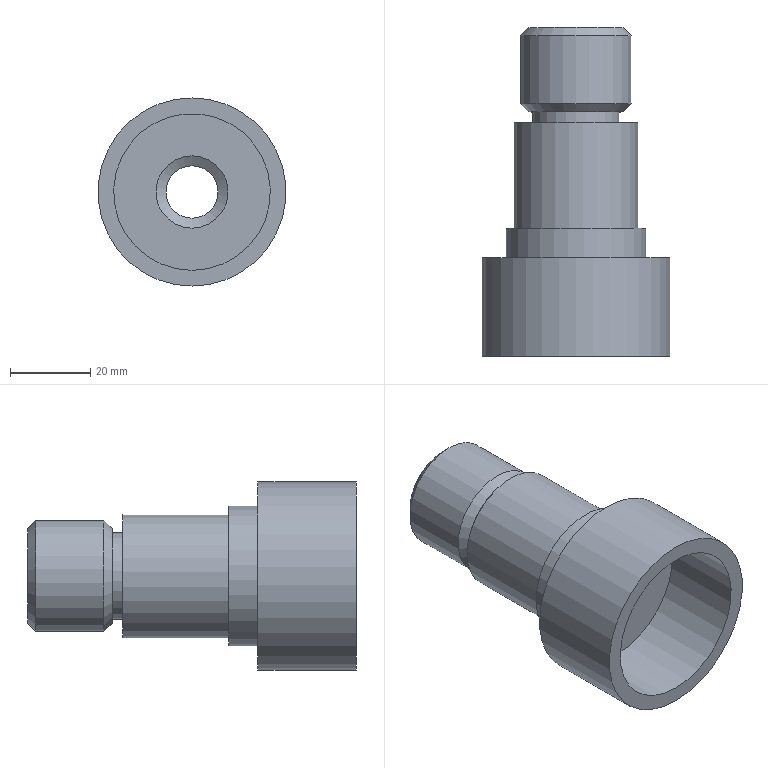Component | NX | VENT_VALVE | 1 solid | 18 faces | box 46.8 x 81.8 x 46.8 mm | volume 45200 mm3 | cylinder 8 | plane 7 | cone 3 | commonest cylinder face diameters 30.8 x1 34.8 x1 46.8 x1 39 x1 13 x1 27.592 x1 21.592 x1 18 x1
STEP:
#1=CARTESIAN_POINT('',(0.,0.,0.));
#2=DIRECTION('',(0.,0.,1.));
#3=DIRECTION('',(1.,0.,0.));
#4=AXIS2_PLACEMENT_3D('',#1,#2,#3);
#5=CARTESIAN_POINT('',(43.195,100.209,-15.4));
#6=VERTEX_POINT('',#5);
#7=CARTESIAN_POINT('',(43.195,100.209,0.));
#8=DIRECTION('',(0.,-1.,0.));
#9=DIRECTION('',(0.,0.,-1.));
#10=AXIS2_PLACEMENT_3D('',#7,#8,#9);
#11=CIRCLE('',#10,15.4);
#12=CARTESIAN_POINT('',(43.195,68.409,0.));
#13=DIRECTION('',(0.,-1.,0.));
#14=DIRECTION('',(0.,0.,-1.));
#15=AXIS2_PLACEMENT_3D('',#12,#13,#14);
#16=CYLINDRICAL_SURFACE('',#15,15.4);
#17=CARTESIAN_POINT('',(0.,-31.8));
#18=DIRECTION('',(1.,0.));
#19=VECTOR('',#18,1.);
#20=LINE('',#17,#19);
#21=(GEOMETRIC_REPRESENTATION_CONTEXT(2)PARAMETRIC_REPRESENTATION_CONTEXT()REPRESENTATION_CONTEXT('',''));
#22=DEFINITIONAL_REPRESENTATION('',(#20),#21);
#23=PCURVE('',#16,#22);
#24=CARTESIAN_POINT('',(27.795,100.209,0.));
#25=DIRECTION('',(0.,-1.,0.));
#26=DIRECTION('',(0.,0.,-1.));
#27=AXIS2_PLACEMENT_3D('',#24,#25,#26);
#28=PLANE('',#27);
#29=CARTESIAN_POINT('',(0.,15.4));
#30=DIRECTION('',(1.,0.));
#31=AXIS2_PLACEMENT_2D('',#29,#30);
#32=CIRCLE('',#31,15.4);
#33=(GEOMETRIC_REPRESENTATION_CONTEXT(2)PARAMETRIC_REPRESENTATION_CONTEXT()REPRESENTATION_CONTEXT('',''));
#34=DEFINITIONAL_REPRESENTATION('',(#32),#33);
#35=PCURVE('',#28,#34);
#36=SURFACE_CURVE('',#11,(#23,#35),.PCURVE_S1.);
#37=EDGE_CURVE('',#6,#6,#36,.T.);
#38=ORIENTED_EDGE('',*,*,#37,.F.);
#39=CARTESIAN_POINT('',(43.195,126.509,-15.4));
#40=VERTEX_POINT('',#39);
#41=CARTESIAN_POINT('',(43.195,126.509,-15.4));
#42=CARTESIAN_POINT('',(43.195,100.209,-15.4));
#43=B_SPLINE_CURVE_WITH_KNOTS('',1,(#41,#42),.UNSPECIFIED.,.F.,.F.,(2,2),(-58.1,-31.8),.PIECEWISE_BEZIER_KNOTS.);
#44=CARTESIAN_POINT('',(0.,0.));
#45=DIRECTION('',(0.,1.));
#46=VECTOR('',#45,1.);
#47=LINE('',#44,#46);
#48=(GEOMETRIC_REPRESENTATION_CONTEXT(2)PARAMETRIC_REPRESENTATION_CONTEXT()REPRESENTATION_CONTEXT('',''));
#49=DEFINITIONAL_REPRESENTATION('',(#47),#48);
#50=PCURVE('',#16,#49);
#51=CARTESIAN_POINT('',(6.283,0.));
#52=DIRECTION('',(0.,1.));
#53=VECTOR('',#52,1.);
#54=LINE('',#51,#53);
#55=(GEOMETRIC_REPRESENTATION_CONTEXT(2)PARAMETRIC_REPRESENTATION_CONTEXT()REPRESENTATION_CONTEXT('',''));
#56=DEFINITIONAL_REPRESENTATION('',(#54),#55);
#57=PCURVE('',#16,#56);
#58=SEAM_CURVE('',#43,(#50,#57),.PCURVE_S1.);
#59=EDGE_CURVE('',#40,#6,#58,.T.);
#60=ORIENTED_EDGE('',*,*,#59,.F.);
#61=CARTESIAN_POINT('',(43.195,126.509,0.));
#62=DIRECTION('',(0.,-1.,0.));
#63=DIRECTION('',(0.,0.,-1.));
#64=AXIS2_PLACEMENT_3D('',#61,#62,#63);
#65=CIRCLE('',#64,15.4);
#66=CARTESIAN_POINT('',(0.,-58.1));
#67=DIRECTION('',(1.,0.));
#68=VECTOR('',#67,1.);
#69=LINE('',#66,#68);
#70=(GEOMETRIC_REPRESENTATION_CONTEXT(2)PARAMETRIC_REPRESENTATION_CONTEXT()REPRESENTATION_CONTEXT('',''));
#71=DEFINITIONAL_REPRESENTATION('',(#69),#70);
#72=PCURVE('',#16,#71);
#73=CARTESIAN_POINT('',(32.399,126.509,0.));
#74=DIRECTION('',(0.,-1.,0.));
#75=DIRECTION('',(0.,0.,-1.));
#76=AXIS2_PLACEMENT_3D('',#73,#74,#75);
#77=PLANE('',#76);
#78=CARTESIAN_POINT('',(0.,10.796));
#79=DIRECTION('',(1.,0.));
#80=AXIS2_PLACEMENT_2D('',#78,#79);
#81=CIRCLE('',#80,15.4);
#82=(GEOMETRIC_REPRESENTATION_CONTEXT(2)PARAMETRIC_REPRESENTATION_CONTEXT()REPRESENTATION_CONTEXT('',''));
#83=DEFINITIONAL_REPRESENTATION('',(#81),#82);
#84=PCURVE('',#77,#83);
#85=SURFACE_CURVE('',#65,(#72,#84),.PCURVE_S1.);
#86=EDGE_CURVE('',#40,#40,#85,.T.);
#87=ORIENTED_EDGE('',*,*,#86,.T.);
#88=ORIENTED_EDGE('',*,*,#59,.T.);
#89=EDGE_LOOP('',(#38,#60,#87,#88));
#90=FACE_BOUND('',#89,.T.);
#91=ADVANCED_FACE('',(#90),#16,.T.);
#92=CARTESIAN_POINT('',(43.195,100.209,-17.4));
#93=VERTEX_POINT('',#92);
#94=CARTESIAN_POINT('',(43.195,100.209,0.));
#95=DIRECTION('',(0.,-1.,0.));
#96=DIRECTION('',(0.,0.,-1.));
#97=AXIS2_PLACEMENT_3D('',#94,#95,#96);
#98=CIRCLE('',#97,17.4);
#99=CARTESIAN_POINT('',(0.,15.4));
#100=DIRECTION('',(1.,0.));
#101=AXIS2_PLACEMENT_2D('',#99,#100);
#102=CIRCLE('',#101,17.4);
#103=(GEOMETRIC_REPRESENTATION_CONTEXT(2)PARAMETRIC_REPRESENTATION_CONTEXT()REPRESENTATION_CONTEXT('',''));
#104=DEFINITIONAL_REPRESENTATION('',(#102),#103);
#105=PCURVE('',#28,#104);
#106=CARTESIAN_POINT('',(43.195,68.409,0.));
#107=DIRECTION('',(0.,-1.,0.));
#108=DIRECTION('',(0.,0.,-1.));
#109=AXIS2_PLACEMENT_3D('',#106,#107,#108);
#110=CYLINDRICAL_SURFACE('',#109,17.4);
#111=CARTESIAN_POINT('',(0.,-31.8));
#112=DIRECTION('',(1.,0.));
#113=VECTOR('',#112,1.);
#114=LINE('',#111,#113);
#115=(GEOMETRIC_REPRESENTATION_CONTEXT(2)PARAMETRIC_REPRESENTATION_CONTEXT()REPRESENTATION_CONTEXT('',''));
#116=DEFINITIONAL_REPRESENTATION('',(#114),#115);
#117=PCURVE('',#110,#116);
#118=SURFACE_CURVE('',#98,(#105,#117),.PCURVE_S1.);
#119=EDGE_CURVE('',#93,#93,#118,.T.);
#120=ORIENTED_EDGE('',*,*,#119,.F.);
#121=EDGE_LOOP('',(#120));
#122=FACE_BOUND('',#121,.T.);
#123=ORIENTED_EDGE('',*,*,#37,.T.);
#124=EDGE_LOOP('',(#123));
#125=FACE_BOUND('',#124,.T.);
#126=ADVANCED_FACE('',(#122,#125),#28,.F.);
#127=CARTESIAN_POINT('',(43.195,92.909,-17.4));
#128=VERTEX_POINT('',#127);
#129=CARTESIAN_POINT('',(43.195,92.909,0.));
#130=DIRECTION('',(0.,-1.,0.));
#131=DIRECTION('',(0.,0.,-1.));
#132=AXIS2_PLACEMENT_3D('',#129,#130,#131);
#133=CIRCLE('',#132,17.4);
#134=CARTESIAN_POINT('',(0.,-24.5));
#135=DIRECTION('',(1.,0.));
#136=VECTOR('',#135,1.);
#137=LINE('',#134,#136);
#138=(GEOMETRIC_REPRESENTATION_CONTEXT(2)PARAMETRIC_REPRESENTATION_CONTEXT()REPRESENTATION_CONTEXT('',''));
#139=DEFINITIONAL_REPRESENTATION('',(#137),#138);
#140=PCURVE('',#110,#139);
#141=CARTESIAN_POINT('',(25.795,92.909,0.));
#142=DIRECTION('',(0.,-1.,0.));
#143=DIRECTION('',(0.,0.,-1.));
#144=AXIS2_PLACEMENT_3D('',#141,#142,#143);
#145=PLANE('',#144);
#146=CARTESIAN_POINT('',(0.,17.4));
#147=DIRECTION('',(1.,0.));
#148=AXIS2_PLACEMENT_2D('',#146,#147);
#149=CIRCLE('',#148,17.4);
#150=(GEOMETRIC_REPRESENTATION_CONTEXT(2)PARAMETRIC_REPRESENTATION_CONTEXT()REPRESENTATION_CONTEXT('',''));
#151=DEFINITIONAL_REPRESENTATION('',(#149),#150);
#152=PCURVE('',#145,#151);
#153=SURFACE_CURVE('',#133,(#140,#152),.PCURVE_S1.);
#154=EDGE_CURVE('',#128,#128,#153,.T.);
#155=ORIENTED_EDGE('',*,*,#154,.F.);
#156=CARTESIAN_POINT('',(43.195,100.209,-17.4));
#157=CARTESIAN_POINT('',(43.195,92.909,-17.4));
#158=B_SPLINE_CURVE_WITH_KNOTS('',1,(#156,#157),.UNSPECIFIED.,.F.,.F.,(2,2),(-31.8,-24.5),.PIECEWISE_BEZIER_KNOTS.);
#159=CARTESIAN_POINT('',(0.,0.));
#160=DIRECTION('',(0.,1.));
#161=VECTOR('',#160,1.);
#162=LINE('',#159,#161);
#163=(GEOMETRIC_REPRESENTATION_CONTEXT(2)PARAMETRIC_REPRESENTATION_CONTEXT()REPRESENTATION_CONTEXT('',''));
#164=DEFINITIONAL_REPRESENTATION('',(#162),#163);
#165=PCURVE('',#110,#164);
#166=CARTESIAN_POINT('',(6.283,0.));
#167=DIRECTION('',(0.,1.));
#168=VECTOR('',#167,1.);
#169=LINE('',#166,#168);
#170=(GEOMETRIC_REPRESENTATION_CONTEXT(2)PARAMETRIC_REPRESENTATION_CONTEXT()REPRESENTATION_CONTEXT('',''));
#171=DEFINITIONAL_REPRESENTATION('',(#169),#170);
#172=PCURVE('',#110,#171);
#173=SEAM_CURVE('',#158,(#165,#172),.PCURVE_S1.);
#174=EDGE_CURVE('',#93,#128,#173,.T.);
#175=ORIENTED_EDGE('',*,*,#174,.F.);
#176=ORIENTED_EDGE('',*,*,#119,.T.);
#177=ORIENTED_EDGE('',*,*,#174,.T.);
#178=EDGE_LOOP('',(#155,#175,#176,#177));
#179=FACE_BOUND('',#178,.T.);
#180=ADVANCED_FACE('',(#179),#110,.T.);
#181=CARTESIAN_POINT('',(43.195,92.909,-23.4));
#182=VERTEX_POINT('',#181);
#183=CARTESIAN_POINT('',(43.195,92.909,0.));
#184=DIRECTION('',(0.,-1.,0.));
#185=DIRECTION('',(0.,0.,-1.));
#186=AXIS2_PLACEMENT_3D('',#183,#184,#185);
#187=CIRCLE('',#186,23.4);
#188=CARTESIAN_POINT('',(0.,17.4));
#189=DIRECTION('',(1.,0.));
#190=AXIS2_PLACEMENT_2D('',#188,#189);
#191=CIRCLE('',#190,23.4);
#192=(GEOMETRIC_REPRESENTATION_CONTEXT(2)PARAMETRIC_REPRESENTATION_CONTEXT()REPRESENTATION_CONTEXT('',''));
#193=DEFINITIONAL_REPRESENTATION('',(#191),#192);
#194=PCURVE('',#145,#193);
#195=CARTESIAN_POINT('',(43.195,68.409,0.));
#196=DIRECTION('',(0.,-1.,0.));
#197=DIRECTION('',(0.,0.,-1.));
#198=AXIS2_PLACEMENT_3D('',#195,#196,#197);
#199=CYLINDRICAL_SURFACE('',#198,23.4);
#200=CARTESIAN_POINT('',(0.,-24.5));
#201=DIRECTION('',(1.,0.));
#202=VECTOR('',#201,1.);
#203=LINE('',#200,#202);
#204=(GEOMETRIC_REPRESENTATION_CONTEXT(2)PARAMETRIC_REPRESENTATION_CONTEXT()REPRESENTATION_CONTEXT('',''));
#205=DEFINITIONAL_REPRESENTATION('',(#203),#204);
#206=PCURVE('',#199,#205);
#207=SURFACE_CURVE('',#187,(#194,#206),.PCURVE_S1.);
#208=EDGE_CURVE('',#182,#182,#207,.T.);
#209=ORIENTED_EDGE('',*,*,#208,.F.);
#210=EDGE_LOOP('',(#209));
#211=FACE_BOUND('',#210,.T.);
#212=ORIENTED_EDGE('',*,*,#154,.T.);
#213=EDGE_LOOP('',(#212));
#214=FACE_BOUND('',#213,.T.);
#215=ADVANCED_FACE('',(#211,#214),#145,.F.);
#216=CARTESIAN_POINT('',(43.195,68.409,-23.4));
#217=VERTEX_POINT('',#216);
#218=CARTESIAN_POINT('',(43.195,68.409,0.));
#219=DIRECTION('',(0.,-1.,0.));
#220=DIRECTION('',(0.,0.,-1.));
#221=AXIS2_PLACEMENT_3D('',#218,#219,#220);
#222=CIRCLE('',#221,23.4);
#223=CARTESIAN_POINT('',(0.,0.));
#224=DIRECTION('',(1.,0.));
#225=VECTOR('',#224,1.);
#226=LINE('',#223,#225);
#227=(GEOMETRIC_REPRESENTATION_CONTEXT(2)PARAMETRIC_REPRESENTATION_CONTEXT()REPRESENTATION_CONTEXT('',''));
#228=DEFINITIONAL_REPRESENTATION('',(#226),#227);
#229=PCURVE('',#199,#228);
#230=CARTESIAN_POINT('',(19.795,68.409,0.));
#231=DIRECTION('',(0.,1.,0.));
#232=DIRECTION('',(0.,0.,1.));
#233=AXIS2_PLACEMENT_3D('',#230,#231,#232);
#234=PLANE('',#233);
#235=CARTESIAN_POINT('',(-23.4,23.4));
#236=CARTESIAN_POINT('',(-23.4,63.93));
#237=CARTESIAN_POINT('',(11.7,43.665));
#238=CARTESIAN_POINT('',(46.8,23.4));
#239=CARTESIAN_POINT('',(11.7,3.135));
#240=CARTESIAN_POINT('',(-23.4,-17.13));
#241=CARTESIAN_POINT('',(-23.4,23.4));
#242=(BOUNDED_CURVE()B_SPLINE_CURVE(2,(#235,#236,#237,#238,#239,#240,#241),.UNSPECIFIED.,.T.,.F.)B_SPLINE_CURVE_WITH_KNOTS((1,2,2,2,2,1),(-2.094,0.,2.094,4.189,6.283,8.378),.UNSPECIFIED.)CURVE()GEOMETRIC_REPRESENTATION_ITEM()RATIONAL_B_SPLINE_CURVE((1.,0.5,1.,0.5,1.,0.5,1.))REPRESENTATION_ITEM(''));
#243=(GEOMETRIC_REPRESENTATION_CONTEXT(2)PARAMETRIC_REPRESENTATION_CONTEXT()REPRESENTATION_CONTEXT('',''));
#244=DEFINITIONAL_REPRESENTATION('',(#242),#243);
#245=PCURVE('',#234,#244);
#246=SURFACE_CURVE('',#222,(#229,#245),.PCURVE_S1.);
#247=EDGE_CURVE('',#217,#217,#246,.T.);
#248=ORIENTED_EDGE('',*,*,#247,.F.);
#249=CARTESIAN_POINT('',(43.195,92.909,-23.4));
#250=CARTESIAN_POINT('',(43.195,68.409,-23.4));
#251=B_SPLINE_CURVE_WITH_KNOTS('',1,(#249,#250),.UNSPECIFIED.,.F.,.F.,(2,2),(-24.5,0.),.PIECEWISE_BEZIER_KNOTS.);
#252=CARTESIAN_POINT('',(0.,0.));
#253=DIRECTION('',(0.,1.));
#254=VECTOR('',#253,1.);
#255=LINE('',#252,#254);
#256=(GEOMETRIC_REPRESENTATION_CONTEXT(2)PARAMETRIC_REPRESENTATION_CONTEXT()REPRESENTATION_CONTEXT('',''));
#257=DEFINITIONAL_REPRESENTATION('',(#255),#256);
#258=PCURVE('',#199,#257);
#259=CARTESIAN_POINT('',(6.283,0.));
#260=DIRECTION('',(0.,1.));
#261=VECTOR('',#260,1.);
#262=LINE('',#259,#261);
#263=(GEOMETRIC_REPRESENTATION_CONTEXT(2)PARAMETRIC_REPRESENTATION_CONTEXT()REPRESENTATION_CONTEXT('',''));
#264=DEFINITIONAL_REPRESENTATION('',(#262),#263);
#265=PCURVE('',#199,#264);
#266=SEAM_CURVE('',#251,(#258,#265),.PCURVE_S1.);
#267=EDGE_CURVE('',#182,#217,#266,.T.);
#268=ORIENTED_EDGE('',*,*,#267,.F.);
#269=ORIENTED_EDGE('',*,*,#208,.T.);
#270=ORIENTED_EDGE('',*,*,#267,.T.);
#271=EDGE_LOOP('',(#248,#268,#269,#270));
#272=FACE_BOUND('',#271,.T.);
#273=ADVANCED_FACE('',(#272),#199,.T.);
#274=CARTESIAN_POINT('',(43.195,68.409,-19.5));
#275=VERTEX_POINT('',#274);
#276=CARTESIAN_POINT('',(43.195,68.409,0.));
#277=DIRECTION('',(0.,-1.,0.));
#278=DIRECTION('',(0.,0.,-1.));
#279=AXIS2_PLACEMENT_3D('',#276,#277,#278);
#280=CIRCLE('',#279,19.5);
#281=CARTESIAN_POINT('',(-19.5,23.4));
#282=CARTESIAN_POINT('',(-19.5,57.175));
#283=CARTESIAN_POINT('',(9.75,40.287));
#284=CARTESIAN_POINT('',(39.,23.4));
#285=CARTESIAN_POINT('',(9.75,6.513));
#286=CARTESIAN_POINT('',(-19.5,-10.375));
#287=CARTESIAN_POINT('',(-19.5,23.4));
#288=(BOUNDED_CURVE()B_SPLINE_CURVE(2,(#281,#282,#283,#284,#285,#286,#287),.UNSPECIFIED.,.T.,.F.)B_SPLINE_CURVE_WITH_KNOTS((1,2,2,2,2,1),(-2.094,0.,2.094,4.189,6.283,8.378),.UNSPECIFIED.)CURVE()GEOMETRIC_REPRESENTATION_ITEM()RATIONAL_B_SPLINE_CURVE((1.,0.5,1.,0.5,1.,0.5,1.))REPRESENTATION_ITEM(''));
#289=(GEOMETRIC_REPRESENTATION_CONTEXT(2)PARAMETRIC_REPRESENTATION_CONTEXT()REPRESENTATION_CONTEXT('',''));
#290=DEFINITIONAL_REPRESENTATION('',(#288),#289);
#291=PCURVE('',#234,#290);
#292=CARTESIAN_POINT('',(43.195,68.409,0.));
#293=DIRECTION('',(0.,-1.,0.));
#294=DIRECTION('',(0.,0.,-1.));
#295=AXIS2_PLACEMENT_3D('',#292,#293,#294);
#296=CYLINDRICAL_SURFACE('',#295,19.5);
#297=CARTESIAN_POINT('',(0.,0.));
#298=DIRECTION('',(1.,0.));
#299=VECTOR('',#298,1.);
#300=LINE('',#297,#299);
#301=(GEOMETRIC_REPRESENTATION_CONTEXT(2)PARAMETRIC_REPRESENTATION_CONTEXT()REPRESENTATION_CONTEXT('',''));
#302=DEFINITIONAL_REPRESENTATION('',(#300),#301);
#303=PCURVE('',#296,#302);
#304=SURFACE_CURVE('',#280,(#291,#303),.PCURVE_S1.);
#305=EDGE_CURVE('',#275,#275,#304,.T.);
#306=ORIENTED_EDGE('',*,*,#305,.F.);
#307=EDGE_LOOP('',(#306));
#308=FACE_BOUND('',#307,.T.);
#309=ORIENTED_EDGE('',*,*,#247,.T.);
#310=EDGE_LOOP('',(#309));
#311=FACE_BOUND('',#310,.T.);
#312=ADVANCED_FACE('',(#308,#311),#234,.F.);
#313=CARTESIAN_POINT('',(43.195,89.109,-19.5));
#314=VERTEX_POINT('',#313);
#315=CARTESIAN_POINT('',(43.195,89.109,0.));
#316=DIRECTION('',(0.,-1.,0.));
#317=DIRECTION('',(0.,0.,-1.));
#318=AXIS2_PLACEMENT_3D('',#315,#316,#317);
#319=CIRCLE('',#318,19.5);
#320=CARTESIAN_POINT('',(0.,-20.7));
#321=DIRECTION('',(1.,0.));
#322=VECTOR('',#321,1.);
#323=LINE('',#320,#322);
#324=(GEOMETRIC_REPRESENTATION_CONTEXT(2)PARAMETRIC_REPRESENTATION_CONTEXT()REPRESENTATION_CONTEXT('',''));
#325=DEFINITIONAL_REPRESENTATION('',(#323),#324);
#326=PCURVE('',#296,#325);
#327=CARTESIAN_POINT('',(23.695,89.109,0.));
#328=DIRECTION('',(0.,1.,0.));
#329=DIRECTION('',(0.,0.,1.));
#330=AXIS2_PLACEMENT_3D('',#327,#328,#329);
#331=PLANE('',#330);
#332=CARTESIAN_POINT('',(-19.5,19.5));
#333=CARTESIAN_POINT('',(-19.5,53.275));
#334=CARTESIAN_POINT('',(9.75,36.387));
#335=CARTESIAN_POINT('',(39.,19.5));
#336=CARTESIAN_POINT('',(9.75,2.613));
#337=CARTESIAN_POINT('',(-19.5,-14.275));
#338=CARTESIAN_POINT('',(-19.5,19.5));
#339=(BOUNDED_CURVE()B_SPLINE_CURVE(2,(#332,#333,#334,#335,#336,#337,#338),.UNSPECIFIED.,.T.,.F.)B_SPLINE_CURVE_WITH_KNOTS((1,2,2,2,2,1),(-2.094,0.,2.094,4.189,6.283,8.378),.UNSPECIFIED.)CURVE()GEOMETRIC_REPRESENTATION_ITEM()RATIONAL_B_SPLINE_CURVE((1.,0.5,1.,0.5,1.,0.5,1.))REPRESENTATION_ITEM(''));
#340=(GEOMETRIC_REPRESENTATION_CONTEXT(2)PARAMETRIC_REPRESENTATION_CONTEXT()REPRESENTATION_CONTEXT('',''));
#341=DEFINITIONAL_REPRESENTATION('',(#339),#340);
#342=PCURVE('',#331,#341);
#343=SURFACE_CURVE('',#319,(#326,#342),.PCURVE_S1.);
#344=EDGE_CURVE('',#314,#314,#343,.T.);
#345=ORIENTED_EDGE('',*,*,#344,.T.);
#346=CARTESIAN_POINT('',(43.195,89.109,-19.5));
#347=CARTESIAN_POINT('',(43.195,68.409,-19.5));
#348=B_SPLINE_CURVE_WITH_KNOTS('',1,(#346,#347),.UNSPECIFIED.,.F.,.F.,(2,2),(-20.7,0.),.PIECEWISE_BEZIER_KNOTS.);
#349=CARTESIAN_POINT('',(6.283,0.));
#350=DIRECTION('',(0.,1.));
#351=VECTOR('',#350,1.);
#352=LINE('',#349,#351);
#353=(GEOMETRIC_REPRESENTATION_CONTEXT(2)PARAMETRIC_REPRESENTATION_CONTEXT()REPRESENTATION_CONTEXT('',''));
#354=DEFINITIONAL_REPRESENTATION('',(#352),#353);
#355=PCURVE('',#296,#354);
#356=CARTESIAN_POINT('',(0.,0.));
#357=DIRECTION('',(0.,1.));
#358=VECTOR('',#357,1.);
#359=LINE('',#356,#358);
#360=(GEOMETRIC_REPRESENTATION_CONTEXT(2)PARAMETRIC_REPRESENTATION_CONTEXT()REPRESENTATION_CONTEXT('',''));
#361=DEFINITIONAL_REPRESENTATION('',(#359),#360);
#362=PCURVE('',#296,#361);
#363=SEAM_CURVE('',#348,(#355,#362),.PCURVE_S1.);
#364=EDGE_CURVE('',#314,#275,#363,.T.);
#365=ORIENTED_EDGE('',*,*,#364,.T.);
#366=ORIENTED_EDGE('',*,*,#305,.F.);
#367=ORIENTED_EDGE('',*,*,#364,.F.);
#368=EDGE_LOOP('',(#345,#365,#366,#367));
#369=FACE_BOUND('',#368,.F.);
#370=ADVANCED_FACE('',(#369),#296,.F.);
#371=CARTESIAN_POINT('',(43.195,89.109,9.));
#372=VERTEX_POINT('',#371);
#373=CARTESIAN_POINT('',(43.195,89.109,0.));
#374=DIRECTION('',(0.,1.,0.));
#375=DIRECTION('',(0.,0.,1.));
#376=AXIS2_PLACEMENT_3D('',#373,#374,#375);
#377=CIRCLE('',#376,9.);
#378=CARTESIAN_POINT('',(0.,19.5));
#379=DIRECTION('',(1.,0.));
#380=AXIS2_PLACEMENT_2D('',#378,#379);
#381=CIRCLE('',#380,9.);
#382=(GEOMETRIC_REPRESENTATION_CONTEXT(2)PARAMETRIC_REPRESENTATION_CONTEXT()REPRESENTATION_CONTEXT('',''));
#383=DEFINITIONAL_REPRESENTATION('',(#381),#382);
#384=PCURVE('',#331,#383);
#385=CARTESIAN_POINT('',(43.195,89.109,0.));
#386=DIRECTION('',(0.,1.,0.));
#387=DIRECTION('',(0.,0.,1.));
#388=AXIS2_PLACEMENT_3D('',#385,#386,#387);
#389=CYLINDRICAL_SURFACE('',#388,9.);
#390=CARTESIAN_POINT('',(0.,0.));
#391=DIRECTION('',(1.,0.));
#392=VECTOR('',#391,1.);
#393=LINE('',#390,#392);
#394=(GEOMETRIC_REPRESENTATION_CONTEXT(2)PARAMETRIC_REPRESENTATION_CONTEXT()REPRESENTATION_CONTEXT('',''));
#395=DEFINITIONAL_REPRESENTATION('',(#393),#394);
#396=PCURVE('',#389,#395);
#397=SURFACE_CURVE('',#377,(#384,#396),.PCURVE_S1.);
#398=EDGE_CURVE('',#372,#372,#397,.T.);
#399=ORIENTED_EDGE('',*,*,#398,.T.);
#400=EDGE_LOOP('',(#399));
#401=FACE_BOUND('',#400,.T.);
#402=ORIENTED_EDGE('',*,*,#344,.T.);
#403=EDGE_LOOP('',(#402));
#404=FACE_BOUND('',#403,.T.);
#405=ADVANCED_FACE('',(#401,#404),#331,.F.);
#406=CARTESIAN_POINT('',(43.195,121.612,-6.5));
#407=VERTEX_POINT('',#406);
#408=CARTESIAN_POINT('',(43.195,121.612,0.));
#409=DIRECTION('',(0.,-1.,0.));
#410=DIRECTION('',(0.,0.,-1.));
#411=AXIS2_PLACEMENT_3D('',#408,#409,#410);
#412=CIRCLE('',#411,6.5);
#413=CARTESIAN_POINT('',(43.195,68.409,0.));
#414=DIRECTION('',(0.,-1.,0.));
#415=DIRECTION('',(0.,0.,-1.));
#416=AXIS2_PLACEMENT_3D('',#413,#414,#415);
#417=CYLINDRICAL_SURFACE('',#416,6.5);
#418=CARTESIAN_POINT('',(0.,-53.202));
#419=DIRECTION('',(1.,0.));
#420=VECTOR('',#419,1.);
#421=LINE('',#418,#420);
#422=(GEOMETRIC_REPRESENTATION_CONTEXT(2)PARAMETRIC_REPRESENTATION_CONTEXT()REPRESENTATION_CONTEXT('',''));
#423=DEFINITIONAL_REPRESENTATION('',(#421),#422);
#424=PCURVE('',#417,#423);
#425=CARTESIAN_POINT('',(43.195,120.109,0.));
#426=DIRECTION('',(0.,-1.,0.));
#427=DIRECTION('',(0.,0.,-1.));
#428=AXIS2_PLACEMENT_3D('',#425,#426,#427);
#429=CONICAL_SURFACE('',#428,9.,1.03);
#430=CARTESIAN_POINT('',(0.,-1.502));
#431=DIRECTION('',(1.,0.));
#432=VECTOR('',#431,1.);
#433=LINE('',#430,#432);
#434=(GEOMETRIC_REPRESENTATION_CONTEXT(2)PARAMETRIC_REPRESENTATION_CONTEXT()REPRESENTATION_CONTEXT('',''));
#435=DEFINITIONAL_REPRESENTATION('',(#433),#434);
#436=PCURVE('',#429,#435);
#437=SURFACE_CURVE('',#412,(#424,#436),.PCURVE_S1.);
#438=EDGE_CURVE('',#407,#407,#437,.T.);
#439=ORIENTED_EDGE('',*,*,#438,.F.);
#440=CARTESIAN_POINT('',(43.195,150.209,-6.5));
#441=VERTEX_POINT('',#440);
#442=CARTESIAN_POINT('',(43.195,150.209,-6.5));
#443=CARTESIAN_POINT('',(43.195,121.612,-6.5));
#444=B_SPLINE_CURVE_WITH_KNOTS('',1,(#442,#443),.UNSPECIFIED.,.F.,.F.,(2,2),(-81.8,-53.202),.PIECEWISE_BEZIER_KNOTS.);
#445=CARTESIAN_POINT('',(0.,0.));
#446=DIRECTION('',(0.,1.));
#447=VECTOR('',#446,1.);
#448=LINE('',#445,#447);
#449=(GEOMETRIC_REPRESENTATION_CONTEXT(2)PARAMETRIC_REPRESENTATION_CONTEXT()REPRESENTATION_CONTEXT('',''));
#450=DEFINITIONAL_REPRESENTATION('',(#448),#449);
#451=PCURVE('',#417,#450);
#452=CARTESIAN_POINT('',(6.283,0.));
#453=DIRECTION('',(0.,1.));
#454=VECTOR('',#453,1.);
#455=LINE('',#452,#454);
#456=(GEOMETRIC_REPRESENTATION_CONTEXT(2)PARAMETRIC_REPRESENTATION_CONTEXT()REPRESENTATION_CONTEXT('',''));
#457=DEFINITIONAL_REPRESENTATION('',(#455),#456);
#458=PCURVE('',#417,#457);
#459=SEAM_CURVE('',#444,(#451,#458),.PCURVE_S1.);
#460=EDGE_CURVE('',#441,#407,#459,.T.);
#461=ORIENTED_EDGE('',*,*,#460,.F.);
#462=CARTESIAN_POINT('',(43.195,150.209,0.));
#463=DIRECTION('',(0.,-1.,0.));
#464=DIRECTION('',(0.,0.,-1.));
#465=AXIS2_PLACEMENT_3D('',#462,#463,#464);
#466=CIRCLE('',#465,6.5);
#467=CARTESIAN_POINT('',(0.,-81.8));
#468=DIRECTION('',(1.,0.));
#469=VECTOR('',#468,1.);
#470=LINE('',#467,#469);
#471=(GEOMETRIC_REPRESENTATION_CONTEXT(2)PARAMETRIC_REPRESENTATION_CONTEXT()REPRESENTATION_CONTEXT('',''));
#472=DEFINITIONAL_REPRESENTATION('',(#470),#471);
#473=PCURVE('',#417,#472);
#474=CARTESIAN_POINT('',(36.695,150.209,0.));
#475=DIRECTION('',(0.,-1.,0.));
#476=DIRECTION('',(0.,0.,-1.));
#477=AXIS2_PLACEMENT_3D('',#474,#475,#476);
#478=PLANE('',#477);
#479=CARTESIAN_POINT('',(0.,6.5));
#480=DIRECTION('',(1.,0.));
#481=AXIS2_PLACEMENT_2D('',#479,#480);
#482=CIRCLE('',#481,6.5);
#483=(GEOMETRIC_REPRESENTATION_CONTEXT(2)PARAMETRIC_REPRESENTATION_CONTEXT()REPRESENTATION_CONTEXT('',''));
#484=DEFINITIONAL_REPRESENTATION('',(#482),#483);
#485=PCURVE('',#478,#484);
#486=SURFACE_CURVE('',#466,(#473,#485),.PCURVE_S1.);
#487=EDGE_CURVE('',#441,#441,#486,.T.);
#488=ORIENTED_EDGE('',*,*,#487,.T.);
#489=ORIENTED_EDGE('',*,*,#460,.T.);
#490=EDGE_LOOP('',(#439,#461,#488,#489));
#491=FACE_BOUND('',#490,.F.);
#492=ADVANCED_FACE('',(#491),#417,.F.);
#493=CARTESIAN_POINT('',(43.195,150.209,-11.796));
#494=VERTEX_POINT('',#493);
#495=CARTESIAN_POINT('',(43.195,150.209,0.));
#496=DIRECTION('',(0.,1.,0.));
#497=DIRECTION('',(0.,0.,-1.));
#498=AXIS2_PLACEMENT_3D('',#495,#496,#497);
#499=CIRCLE('',#498,11.796);
#500=CARTESIAN_POINT('',(11.796,6.5));
#501=CARTESIAN_POINT('',(11.796,-13.931));
#502=CARTESIAN_POINT('',(-5.898,-3.716));
#503=CARTESIAN_POINT('',(-23.592,6.5));
#504=CARTESIAN_POINT('',(-5.898,16.716));
#505=CARTESIAN_POINT('',(11.796,26.931));
#506=CARTESIAN_POINT('',(11.796,6.5));
#507=(BOUNDED_CURVE()B_SPLINE_CURVE(2,(#500,#501,#502,#503,#504,#505,#506),.UNSPECIFIED.,.T.,.F.)B_SPLINE_CURVE_WITH_KNOTS((1,2,2,2,2,1),(-2.094,0.,2.094,4.189,6.283,8.378),.UNSPECIFIED.)CURVE()GEOMETRIC_REPRESENTATION_ITEM()RATIONAL_B_SPLINE_CURVE((1.,0.5,1.,0.5,1.,0.5,1.))REPRESENTATION_ITEM(''));
#508=(GEOMETRIC_REPRESENTATION_CONTEXT(2)PARAMETRIC_REPRESENTATION_CONTEXT()REPRESENTATION_CONTEXT('',''));
#509=DEFINITIONAL_REPRESENTATION('',(#507),#508);
#510=PCURVE('',#478,#509);
#511=CARTESIAN_POINT('',(43.195,148.209,0.));
#512=DIRECTION('',(0.,-1.,0.));
#513=DIRECTION('',(0.,0.,-1.));
#514=AXIS2_PLACEMENT_3D('',#511,#512,#513);
#515=CONICAL_SURFACE('',#514,13.796,0.7854);
#516=CARTESIAN_POINT('',(6.283,-2.));
#517=DIRECTION('',(-1.,0.));
#518=VECTOR('',#517,1.);
#519=LINE('',#516,#518);
#520=(GEOMETRIC_REPRESENTATION_CONTEXT(2)PARAMETRIC_REPRESENTATION_CONTEXT()REPRESENTATION_CONTEXT('',''));
#521=DEFINITIONAL_REPRESENTATION('',(#519),#520);
#522=PCURVE('',#515,#521);
#523=SURFACE_CURVE('',#499,(#510,#522),.PCURVE_S1.);
#524=EDGE_CURVE('',#494,#494,#523,.T.);
#525=ORIENTED_EDGE('',*,*,#524,.T.);
#526=EDGE_LOOP('',(#525));
#527=FACE_BOUND('',#526,.T.);
#528=ORIENTED_EDGE('',*,*,#487,.T.);
#529=EDGE_LOOP('',(#528));
#530=FACE_BOUND('',#529,.T.);
#531=ADVANCED_FACE('',(#527,#530),#478,.F.);
#532=CARTESIAN_POINT('',(43.195,131.209,13.796));
#533=VERTEX_POINT('',#532);
#534=CARTESIAN_POINT('',(43.195,131.209,-13.796));
#535=VERTEX_POINT('',#534);
#536=CARTESIAN_POINT('',(43.195,131.209,0.));
#537=DIRECTION('',(0.,1.,0.));
#538=DIRECTION('',(0.,0.,1.));
#539=AXIS2_PLACEMENT_3D('',#536,#537,#538);
#540=CIRCLE('',#539,13.796);
#541=CARTESIAN_POINT('',(43.195,68.409,0.));
#542=DIRECTION('',(0.,-1.,0.));
#543=DIRECTION('',(0.,0.,-1.));
#544=AXIS2_PLACEMENT_3D('',#541,#542,#543);
#545=CYLINDRICAL_SURFACE('',#544,13.796);
#546=CARTESIAN_POINT('',(3.142,-62.8));
#547=DIRECTION('',(-1.,0.));
#548=VECTOR('',#547,1.);
#549=LINE('',#546,#548);
#550=(GEOMETRIC_REPRESENTATION_CONTEXT(2)PARAMETRIC_REPRESENTATION_CONTEXT()REPRESENTATION_CONTEXT('',''));
#551=DEFINITIONAL_REPRESENTATION('',(#549),#550);
#552=PCURVE('',#545,#551);
#553=CARTESIAN_POINT('',(43.195,129.209,0.));
#554=DIRECTION('',(0.,1.,0.));
#555=DIRECTION('',(0.,0.,1.));
#556=AXIS2_PLACEMENT_3D('',#553,#554,#555);
#557=CONICAL_SURFACE('',#556,11.796,0.7854);
#558=CARTESIAN_POINT('',(0.,2.));
#559=DIRECTION('',(1.,0.));
#560=VECTOR('',#559,1.);
#561=LINE('',#558,#560);
#562=(GEOMETRIC_REPRESENTATION_CONTEXT(2)PARAMETRIC_REPRESENTATION_CONTEXT()REPRESENTATION_CONTEXT('',''));
#563=DEFINITIONAL_REPRESENTATION('',(#561),#562);
#564=PCURVE('',#557,#563);
#565=SURFACE_CURVE('',#540,(#552,#564),.PCURVE_S1.);
#566=EDGE_CURVE('',#533,#535,#565,.T.);
#567=ORIENTED_EDGE('',*,*,#566,.T.);
#568=CARTESIAN_POINT('',(43.195,148.209,-13.796));
#569=VERTEX_POINT('',#568);
#570=CARTESIAN_POINT('',(43.195,148.209,-13.796));
#571=CARTESIAN_POINT('',(43.195,131.209,-13.796));
#572=B_SPLINE_CURVE_WITH_KNOTS('',1,(#570,#571),.UNSPECIFIED.,.F.,.F.,(2,2),(-79.8,-62.8),.PIECEWISE_BEZIER_KNOTS.);
#573=CARTESIAN_POINT('',(0.,0.));
#574=DIRECTION('',(0.,1.));
#575=VECTOR('',#574,1.);
#576=LINE('',#573,#575);
#577=(GEOMETRIC_REPRESENTATION_CONTEXT(2)PARAMETRIC_REPRESENTATION_CONTEXT()REPRESENTATION_CONTEXT('',''));
#578=DEFINITIONAL_REPRESENTATION('',(#576),#577);
#579=PCURVE('',#545,#578);
#580=CARTESIAN_POINT('',(6.283,0.));
#581=DIRECTION('',(0.,1.));
#582=VECTOR('',#581,1.);
#583=LINE('',#580,#582);
#584=(GEOMETRIC_REPRESENTATION_CONTEXT(2)PARAMETRIC_REPRESENTATION_CONTEXT()REPRESENTATION_CONTEXT('',''));
#585=DEFINITIONAL_REPRESENTATION('',(#583),#584);
#586=PCURVE('',#545,#585);
#587=SEAM_CURVE('',#572,(#579,#586),.PCURVE_S1.);
#588=EDGE_CURVE('',#569,#535,#587,.T.);
#589=ORIENTED_EDGE('',*,*,#588,.F.);
#590=CARTESIAN_POINT('',(43.195,148.209,0.));
#591=DIRECTION('',(0.,-1.,0.));
#592=DIRECTION('',(0.,0.,-1.));
#593=AXIS2_PLACEMENT_3D('',#590,#591,#592);
#594=CIRCLE('',#593,13.796);
#595=CARTESIAN_POINT('',(0.,-79.8));
#596=DIRECTION('',(1.,0.));
#597=VECTOR('',#596,1.);
#598=LINE('',#595,#597);
#599=(GEOMETRIC_REPRESENTATION_CONTEXT(2)PARAMETRIC_REPRESENTATION_CONTEXT()REPRESENTATION_CONTEXT('',''));
#600=DEFINITIONAL_REPRESENTATION('',(#598),#599);
#601=PCURVE('',#545,#600);
#602=CARTESIAN_POINT('',(0.,0.));
#603=DIRECTION('',(1.,0.));
#604=VECTOR('',#603,1.);
#605=LINE('',#602,#604);
#606=(GEOMETRIC_REPRESENTATION_CONTEXT(2)PARAMETRIC_REPRESENTATION_CONTEXT()REPRESENTATION_CONTEXT('',''));
#607=DEFINITIONAL_REPRESENTATION('',(#605),#606);
#608=PCURVE('',#515,#607);
#609=SURFACE_CURVE('',#594,(#601,#608),.PCURVE_S1.);
#610=EDGE_CURVE('',#569,#569,#609,.T.);
#611=ORIENTED_EDGE('',*,*,#610,.T.);
#612=ORIENTED_EDGE('',*,*,#588,.T.);
#613=CARTESIAN_POINT('',(43.195,131.209,0.));
#614=DIRECTION('',(0.,1.,0.));
#615=DIRECTION('',(0.,0.,1.));
#616=AXIS2_PLACEMENT_3D('',#613,#614,#615);
#617=CIRCLE('',#616,13.796);
#618=CARTESIAN_POINT('',(9.425,-62.8));
#619=DIRECTION('',(-1.,0.));
#620=VECTOR('',#619,1.);
#621=LINE('',#618,#620);
#622=(GEOMETRIC_REPRESENTATION_CONTEXT(2)PARAMETRIC_REPRESENTATION_CONTEXT()REPRESENTATION_CONTEXT('',''));
#623=DEFINITIONAL_REPRESENTATION('',(#621),#622);
#624=PCURVE('',#545,#623);
#625=CARTESIAN_POINT('',(0.,2.));
#626=DIRECTION('',(1.,0.));
#627=VECTOR('',#626,1.);
#628=LINE('',#625,#627);
#629=(GEOMETRIC_REPRESENTATION_CONTEXT(2)PARAMETRIC_REPRESENTATION_CONTEXT()REPRESENTATION_CONTEXT('',''));
#630=DEFINITIONAL_REPRESENTATION('',(#628),#629);
#631=PCURVE('',#557,#630);
#632=SURFACE_CURVE('',#617,(#624,#631),.PCURVE_S1.);
#633=EDGE_CURVE('',#535,#533,#632,.T.);
#634=ORIENTED_EDGE('',*,*,#633,.T.);
#635=EDGE_LOOP('',(#567,#589,#611,#612,#634));
#636=FACE_BOUND('',#635,.T.);
#637=ADVANCED_FACE('',(#636),#545,.T.);
#638=CARTESIAN_POINT('',(43.195,129.209,11.796));
#639=VERTEX_POINT('',#638);
#640=CARTESIAN_POINT('',(43.195,129.209,0.));
#641=DIRECTION('',(0.,-1.,0.));
#642=DIRECTION('',(0.,0.,1.));
#643=AXIS2_PLACEMENT_3D('',#640,#641,#642);
#644=CIRCLE('',#643,11.796);
#645=CARTESIAN_POINT('',(29.399,129.209,0.));
#646=DIRECTION('',(0.,1.,0.));
#647=DIRECTION('',(0.,0.,1.));
#648=AXIS2_PLACEMENT_3D('',#645,#646,#647);
#649=PLANE('',#648);
#650=CARTESIAN_POINT('',(11.796,13.796));
#651=CARTESIAN_POINT('',(11.796,-6.635));
#652=CARTESIAN_POINT('',(-5.898,3.58));
#653=CARTESIAN_POINT('',(-23.592,13.796));
#654=CARTESIAN_POINT('',(-5.898,24.011));
#655=CARTESIAN_POINT('',(11.796,34.227));
#656=CARTESIAN_POINT('',(11.796,13.796));
#657=(BOUNDED_CURVE()B_SPLINE_CURVE(2,(#650,#651,#652,#653,#654,#655,#656),.UNSPECIFIED.,.T.,.F.)B_SPLINE_CURVE_WITH_KNOTS((1,2,2,2,2,1),(-2.094,0.,2.094,4.189,6.283,8.378),.UNSPECIFIED.)CURVE()GEOMETRIC_REPRESENTATION_ITEM()RATIONAL_B_SPLINE_CURVE((1.,0.5,1.,0.5,1.,0.5,1.))REPRESENTATION_ITEM(''));
#658=(GEOMETRIC_REPRESENTATION_CONTEXT(2)PARAMETRIC_REPRESENTATION_CONTEXT()REPRESENTATION_CONTEXT('',''));
#659=DEFINITIONAL_REPRESENTATION('',(#657),#658);
#660=PCURVE('',#649,#659);
#661=CARTESIAN_POINT('',(6.283,0.));
#662=DIRECTION('',(-1.,0.));
#663=VECTOR('',#662,1.);
#664=LINE('',#661,#663);
#665=(GEOMETRIC_REPRESENTATION_CONTEXT(2)PARAMETRIC_REPRESENTATION_CONTEXT()REPRESENTATION_CONTEXT('',''));
#666=DEFINITIONAL_REPRESENTATION('',(#664),#665);
#667=PCURVE('',#557,#666);
#668=SURFACE_CURVE('',#644,(#660,#667),.PCURVE_S1.);
#669=EDGE_CURVE('',#639,#639,#668,.T.);
#670=ORIENTED_EDGE('',*,*,#669,.T.);
#671=EDGE_LOOP('',(#670));
#672=FACE_BOUND('',#671,.T.);
#673=CARTESIAN_POINT('',(43.195,129.209,-10.796));
#674=VERTEX_POINT('',#673);
#675=CARTESIAN_POINT('',(43.195,129.209,0.));
#676=DIRECTION('',(0.,-1.,0.));
#677=DIRECTION('',(0.,0.,-1.));
#678=AXIS2_PLACEMENT_3D('',#675,#676,#677);
#679=CIRCLE('',#678,10.796);
#680=CARTESIAN_POINT('',(-10.796,13.796));
#681=CARTESIAN_POINT('',(-10.796,32.495));
#682=CARTESIAN_POINT('',(5.398,23.145));
#683=CARTESIAN_POINT('',(21.592,13.796));
#684=CARTESIAN_POINT('',(5.398,4.446));
#685=CARTESIAN_POINT('',(-10.796,-4.903));
#686=CARTESIAN_POINT('',(-10.796,13.796));
#687=(BOUNDED_CURVE()B_SPLINE_CURVE(2,(#680,#681,#682,#683,#684,#685,#686),.UNSPECIFIED.,.T.,.F.)B_SPLINE_CURVE_WITH_KNOTS((1,2,2,2,2,1),(-2.094,0.,2.094,4.189,6.283,8.378),.UNSPECIFIED.)CURVE()GEOMETRIC_REPRESENTATION_ITEM()RATIONAL_B_SPLINE_CURVE((1.,0.5,1.,0.5,1.,0.5,1.))REPRESENTATION_ITEM(''));
#688=(GEOMETRIC_REPRESENTATION_CONTEXT(2)PARAMETRIC_REPRESENTATION_CONTEXT()REPRESENTATION_CONTEXT('',''));
#689=DEFINITIONAL_REPRESENTATION('',(#687),#688);
#690=PCURVE('',#649,#689);
#691=CARTESIAN_POINT('',(43.195,68.409,0.));
#692=DIRECTION('',(0.,-1.,0.));
#693=DIRECTION('',(0.,0.,-1.));
#694=AXIS2_PLACEMENT_3D('',#691,#692,#693);
#695=CYLINDRICAL_SURFACE('',#694,10.796);
#696=CARTESIAN_POINT('',(0.,-60.8));
#697=DIRECTION('',(1.,0.));
#698=VECTOR('',#697,1.);
#699=LINE('',#696,#698);
#700=(GEOMETRIC_REPRESENTATION_CONTEXT(2)PARAMETRIC_REPRESENTATION_CONTEXT()REPRESENTATION_CONTEXT('',''));
#701=DEFINITIONAL_REPRESENTATION('',(#699),#700);
#702=PCURVE('',#695,#701);
#703=SURFACE_CURVE('',#679,(#690,#702),.PCURVE_S1.);
#704=EDGE_CURVE('',#674,#674,#703,.T.);
#705=ORIENTED_EDGE('',*,*,#704,.F.);
#706=EDGE_LOOP('',(#705));
#707=FACE_BOUND('',#706,.T.);
#708=ADVANCED_FACE('',(#672,#707),#649,.F.);
#709=CARTESIAN_POINT('',(43.195,126.509,-10.796));
#710=VERTEX_POINT('',#709);
#711=CARTESIAN_POINT('',(43.195,126.509,0.));
#712=DIRECTION('',(0.,-1.,0.));
#713=DIRECTION('',(0.,0.,-1.));
#714=AXIS2_PLACEMENT_3D('',#711,#712,#713);
#715=CIRCLE('',#714,10.796);
#716=CARTESIAN_POINT('',(0.,-58.1));
#717=DIRECTION('',(1.,0.));
#718=VECTOR('',#717,1.);
#719=LINE('',#716,#718);
#720=(GEOMETRIC_REPRESENTATION_CONTEXT(2)PARAMETRIC_REPRESENTATION_CONTEXT()REPRESENTATION_CONTEXT('',''));
#721=DEFINITIONAL_REPRESENTATION('',(#719),#720);
#722=PCURVE('',#695,#721);
#723=CARTESIAN_POINT('',(0.,10.796));
#724=DIRECTION('',(1.,0.));
#725=AXIS2_PLACEMENT_2D('',#723,#724);
#726=CIRCLE('',#725,10.796);
#727=(GEOMETRIC_REPRESENTATION_CONTEXT(2)PARAMETRIC_REPRESENTATION_CONTEXT()REPRESENTATION_CONTEXT('',''));
#728=DEFINITIONAL_REPRESENTATION('',(#726),#727);
#729=PCURVE('',#77,#728);
#730=SURFACE_CURVE('',#715,(#722,#729),.PCURVE_S1.);
#731=EDGE_CURVE('',#710,#710,#730,.T.);
#732=ORIENTED_EDGE('',*,*,#731,.F.);
#733=CARTESIAN_POINT('',(43.195,129.209,-10.796));
#734=CARTESIAN_POINT('',(43.195,126.509,-10.796));
#735=B_SPLINE_CURVE_WITH_KNOTS('',1,(#733,#734),.UNSPECIFIED.,.F.,.F.,(2,2),(-60.8,-58.1),.PIECEWISE_BEZIER_KNOTS.);
#736=CARTESIAN_POINT('',(0.,0.));
#737=DIRECTION('',(0.,1.));
#738=VECTOR('',#737,1.);
#739=LINE('',#736,#738);
#740=(GEOMETRIC_REPRESENTATION_CONTEXT(2)PARAMETRIC_REPRESENTATION_CONTEXT()REPRESENTATION_CONTEXT('',''));
#741=DEFINITIONAL_REPRESENTATION('',(#739),#740);
#742=PCURVE('',#695,#741);
#743=CARTESIAN_POINT('',(6.283,0.));
#744=DIRECTION('',(0.,1.));
#745=VECTOR('',#744,1.);
#746=LINE('',#743,#745);
#747=(GEOMETRIC_REPRESENTATION_CONTEXT(2)PARAMETRIC_REPRESENTATION_CONTEXT()REPRESENTATION_CONTEXT('',''));
#748=DEFINITIONAL_REPRESENTATION('',(#746),#747);
#749=PCURVE('',#695,#748);
#750=SEAM_CURVE('',#735,(#742,#749),.PCURVE_S1.);
#751=EDGE_CURVE('',#674,#710,#750,.T.);
#752=ORIENTED_EDGE('',*,*,#751,.F.);
#753=ORIENTED_EDGE('',*,*,#704,.T.);
#754=ORIENTED_EDGE('',*,*,#751,.T.);
#755=EDGE_LOOP('',(#732,#752,#753,#754));
#756=FACE_BOUND('',#755,.T.);
#757=ADVANCED_FACE('',(#756),#695,.T.);
#758=ORIENTED_EDGE('',*,*,#86,.F.);
#759=EDGE_LOOP('',(#758));
#760=FACE_BOUND('',#759,.T.);
#761=ORIENTED_EDGE('',*,*,#731,.T.);
#762=EDGE_LOOP('',(#761));
#763=FACE_BOUND('',#762,.T.);
#764=ADVANCED_FACE('',(#760,#763),#77,.F.);
#765=CARTESIAN_POINT('',(43.195,120.109,-9.));
#766=VERTEX_POINT('',#765);
#767=CARTESIAN_POINT('',(43.195,120.109,9.));
#768=VERTEX_POINT('',#767);
#769=CARTESIAN_POINT('',(43.195,120.109,0.));
#770=DIRECTION('',(0.,-1.,0.));
#771=DIRECTION('',(0.,0.,1.));
#772=AXIS2_PLACEMENT_3D('',#769,#770,#771);
#773=CIRCLE('',#772,9.);
#774=CARTESIAN_POINT('',(-3.142,0.));
#775=DIRECTION('',(1.,0.));
#776=VECTOR('',#775,1.);
#777=LINE('',#774,#776);
#778=(GEOMETRIC_REPRESENTATION_CONTEXT(2)PARAMETRIC_REPRESENTATION_CONTEXT()REPRESENTATION_CONTEXT('',''));
#779=DEFINITIONAL_REPRESENTATION('',(#777),#778);
#780=PCURVE('',#429,#779);
#781=CARTESIAN_POINT('',(6.283,31.));
#782=DIRECTION('',(-1.,0.));
#783=VECTOR('',#782,1.);
#784=LINE('',#781,#783);
#785=(GEOMETRIC_REPRESENTATION_CONTEXT(2)PARAMETRIC_REPRESENTATION_CONTEXT()REPRESENTATION_CONTEXT('',''));
#786=DEFINITIONAL_REPRESENTATION('',(#784),#785);
#787=PCURVE('',#389,#786);
#788=SURFACE_CURVE('',#773,(#780,#787),.PCURVE_S1.);
#789=EDGE_CURVE('',#766,#768,#788,.T.);
#790=ORIENTED_EDGE('',*,*,#789,.F.);
#791=CARTESIAN_POINT('',(43.195,121.612,-6.5));
#792=CARTESIAN_POINT('',(43.195,120.109,-9.));
#793=B_SPLINE_CURVE_WITH_KNOTS('',1,(#791,#792),.UNSPECIFIED.,.F.,.F.,(2,2),(-2.917,0.),.PIECEWISE_BEZIER_KNOTS.);
#794=CARTESIAN_POINT('',(0.,0.));
#795=DIRECTION('',(0.,1.));
#796=VECTOR('',#795,1.);
#797=LINE('',#794,#796);
#798=(GEOMETRIC_REPRESENTATION_CONTEXT(2)PARAMETRIC_REPRESENTATION_CONTEXT()REPRESENTATION_CONTEXT('',''));
#799=DEFINITIONAL_REPRESENTATION('',(#797),#798);
#800=PCURVE('',#429,#799);
#801=CARTESIAN_POINT('',(6.283,0.));
#802=DIRECTION('',(0.,1.));
#803=VECTOR('',#802,1.);
#804=LINE('',#801,#803);
#805=(GEOMETRIC_REPRESENTATION_CONTEXT(2)PARAMETRIC_REPRESENTATION_CONTEXT()REPRESENTATION_CONTEXT('',''));
#806=DEFINITIONAL_REPRESENTATION('',(#804),#805);
#807=PCURVE('',#429,#806);
#808=SEAM_CURVE('',#793,(#800,#807),.PCURVE_S1.);
#809=EDGE_CURVE('',#407,#766,#808,.T.);
#810=ORIENTED_EDGE('',*,*,#809,.F.);
#811=ORIENTED_EDGE('',*,*,#438,.T.);
#812=ORIENTED_EDGE('',*,*,#809,.T.);
#813=CARTESIAN_POINT('',(43.195,120.109,0.));
#814=DIRECTION('',(0.,-1.,0.));
#815=DIRECTION('',(0.,0.,1.));
#816=AXIS2_PLACEMENT_3D('',#813,#814,#815);
#817=CIRCLE('',#816,9.);
#818=CARTESIAN_POINT('',(3.142,0.));
#819=DIRECTION('',(1.,0.));
#820=VECTOR('',#819,1.);
#821=LINE('',#818,#820);
#822=(GEOMETRIC_REPRESENTATION_CONTEXT(2)PARAMETRIC_REPRESENTATION_CONTEXT()REPRESENTATION_CONTEXT('',''));
#823=DEFINITIONAL_REPRESENTATION('',(#821),#822);
#824=PCURVE('',#429,#823);
#825=CARTESIAN_POINT('',(6.283,31.));
#826=DIRECTION('',(-1.,0.));
#827=VECTOR('',#826,1.);
#828=LINE('',#825,#827);
#829=(GEOMETRIC_REPRESENTATION_CONTEXT(2)PARAMETRIC_REPRESENTATION_CONTEXT()REPRESENTATION_CONTEXT('',''));
#830=DEFINITIONAL_REPRESENTATION('',(#828),#829);
#831=PCURVE('',#389,#830);
#832=SURFACE_CURVE('',#817,(#824,#831),.PCURVE_S1.);
#833=EDGE_CURVE('',#768,#766,#832,.T.);
#834=ORIENTED_EDGE('',*,*,#833,.F.);
#835=EDGE_LOOP('',(#790,#810,#811,#812,#834));
#836=FACE_BOUND('',#835,.F.);
#837=ADVANCED_FACE('',(#836),#429,.F.);
#838=ORIENTED_EDGE('',*,*,#789,.T.);
#839=CARTESIAN_POINT('',(43.195,89.109,9.));
#840=CARTESIAN_POINT('',(43.195,120.109,9.));
#841=B_SPLINE_CURVE_WITH_KNOTS('',1,(#839,#840),.UNSPECIFIED.,.F.,.F.,(2,2),(0.,31.),.PIECEWISE_BEZIER_KNOTS.);
#842=CARTESIAN_POINT('',(0.,0.));
#843=DIRECTION('',(0.,1.));
#844=VECTOR('',#843,1.);
#845=LINE('',#842,#844);
#846=(GEOMETRIC_REPRESENTATION_CONTEXT(2)PARAMETRIC_REPRESENTATION_CONTEXT()REPRESENTATION_CONTEXT('',''));
#847=DEFINITIONAL_REPRESENTATION('',(#845),#846);
#848=PCURVE('',#389,#847);
#849=CARTESIAN_POINT('',(6.283,0.));
#850=DIRECTION('',(0.,1.));
#851=VECTOR('',#850,1.);
#852=LINE('',#849,#851);
#853=(GEOMETRIC_REPRESENTATION_CONTEXT(2)PARAMETRIC_REPRESENTATION_CONTEXT()REPRESENTATION_CONTEXT('',''));
#854=DEFINITIONAL_REPRESENTATION('',(#852),#853);
#855=PCURVE('',#389,#854);
#856=SEAM_CURVE('',#841,(#848,#855),.PCURVE_S1.);
#857=EDGE_CURVE('',#372,#768,#856,.T.);
#858=ORIENTED_EDGE('',*,*,#857,.F.);
#859=ORIENTED_EDGE('',*,*,#398,.T.);
#860=ORIENTED_EDGE('',*,*,#857,.T.);
#861=ORIENTED_EDGE('',*,*,#833,.T.);
#862=EDGE_LOOP('',(#838,#858,#859,#860,#861));
#863=FACE_BOUND('',#862,.F.);
#864=ADVANCED_FACE('',(#863),#389,.F.);
#865=ORIENTED_EDGE('',*,*,#566,.F.);
#866=CARTESIAN_POINT('',(43.195,129.209,11.796));
#867=CARTESIAN_POINT('',(43.195,131.209,13.796));
#868=B_SPLINE_CURVE_WITH_KNOTS('',1,(#866,#867),.UNSPECIFIED.,.F.,.F.,(2,2),(0.,2.828),.PIECEWISE_BEZIER_KNOTS.);
#869=CARTESIAN_POINT('',(0.,0.));
#870=DIRECTION('',(0.,1.));
#871=VECTOR('',#870,1.);
#872=LINE('',#869,#871);
#873=(GEOMETRIC_REPRESENTATION_CONTEXT(2)PARAMETRIC_REPRESENTATION_CONTEXT()REPRESENTATION_CONTEXT('',''));
#874=DEFINITIONAL_REPRESENTATION('',(#872),#873);
#875=PCURVE('',#557,#874);
#876=CARTESIAN_POINT('',(6.283,0.));
#877=DIRECTION('',(0.,1.));
#878=VECTOR('',#877,1.);
#879=LINE('',#876,#878);
#880=(GEOMETRIC_REPRESENTATION_CONTEXT(2)PARAMETRIC_REPRESENTATION_CONTEXT()REPRESENTATION_CONTEXT('',''));
#881=DEFINITIONAL_REPRESENTATION('',(#879),#880);
#882=PCURVE('',#557,#881);
#883=SEAM_CURVE('',#868,(#875,#882),.PCURVE_S1.);
#884=EDGE_CURVE('',#639,#533,#883,.T.);
#885=ORIENTED_EDGE('',*,*,#884,.F.);
#886=ORIENTED_EDGE('',*,*,#669,.F.);
#887=ORIENTED_EDGE('',*,*,#884,.T.);
#888=ORIENTED_EDGE('',*,*,#633,.F.);
#889=EDGE_LOOP('',(#865,#885,#886,#887,#888));
#890=FACE_BOUND('',#889,.T.);
#891=ADVANCED_FACE('',(#890),#557,.T.);
#892=ORIENTED_EDGE('',*,*,#524,.F.);
#893=CARTESIAN_POINT('',(43.195,150.209,-11.796));
#894=CARTESIAN_POINT('',(43.195,148.209,-13.796));
#895=B_SPLINE_CURVE_WITH_KNOTS('',1,(#893,#894),.UNSPECIFIED.,.F.,.F.,(2,2),(-2.828,0.),.PIECEWISE_BEZIER_KNOTS.);
#896=CARTESIAN_POINT('',(6.283,0.));
#897=DIRECTION('',(0.,1.));
#898=VECTOR('',#897,1.);
#899=LINE('',#896,#898);
#900=(GEOMETRIC_REPRESENTATION_CONTEXT(2)PARAMETRIC_REPRESENTATION_CONTEXT()REPRESENTATION_CONTEXT('',''));
#901=DEFINITIONAL_REPRESENTATION('',(#899),#900);
#902=PCURVE('',#515,#901);
#903=CARTESIAN_POINT('',(0.,0.));
#904=DIRECTION('',(0.,1.));
#905=VECTOR('',#904,1.);
#906=LINE('',#903,#905);
#907=(GEOMETRIC_REPRESENTATION_CONTEXT(2)PARAMETRIC_REPRESENTATION_CONTEXT()REPRESENTATION_CONTEXT('',''));
#908=DEFINITIONAL_REPRESENTATION('',(#906),#907);
#909=PCURVE('',#515,#908);
#910=SEAM_CURVE('',#895,(#902,#909),.PCURVE_S1.);
#911=EDGE_CURVE('',#494,#569,#910,.T.);
#912=ORIENTED_EDGE('',*,*,#911,.T.);
#913=ORIENTED_EDGE('',*,*,#610,.F.);
#914=ORIENTED_EDGE('',*,*,#911,.F.);
#915=EDGE_LOOP('',(#892,#912,#913,#914));
#916=FACE_BOUND('',#915,.T.);
#917=ADVANCED_FACE('',(#916),#515,.T.);
#918=CLOSED_SHELL('',(#91,#126,#180,#215,#273,#312,#370,#405,#492,#531,#637,#708,#757,#764,#837,#864,#891,#917));
#919=MANIFOLD_SOLID_BREP('',#918);
#920=(LENGTH_UNIT()NAMED_UNIT(*)SI_UNIT(.MILLI.,.METRE.));
#921=UNCERTAINTY_MEASURE_WITH_UNIT(LENGTH_MEASURE(0.00001),#920,'','');
#922=(NAMED_UNIT(*)PLANE_ANGLE_UNIT()SI_UNIT($,.RADIAN.));
#923=(NAMED_UNIT(*)SI_UNIT($,.STERADIAN.)SOLID_ANGLE_UNIT());
#924=(GEOMETRIC_REPRESENTATION_CONTEXT(3)GLOBAL_UNCERTAINTY_ASSIGNED_CONTEXT((#921))GLOBAL_UNIT_ASSIGNED_CONTEXT((#920,#922,#923))REPRESENTATION_CONTEXT('',''));
#925=ADVANCED_BREP_SHAPE_REPRESENTATION('',(#4,#919),#924);